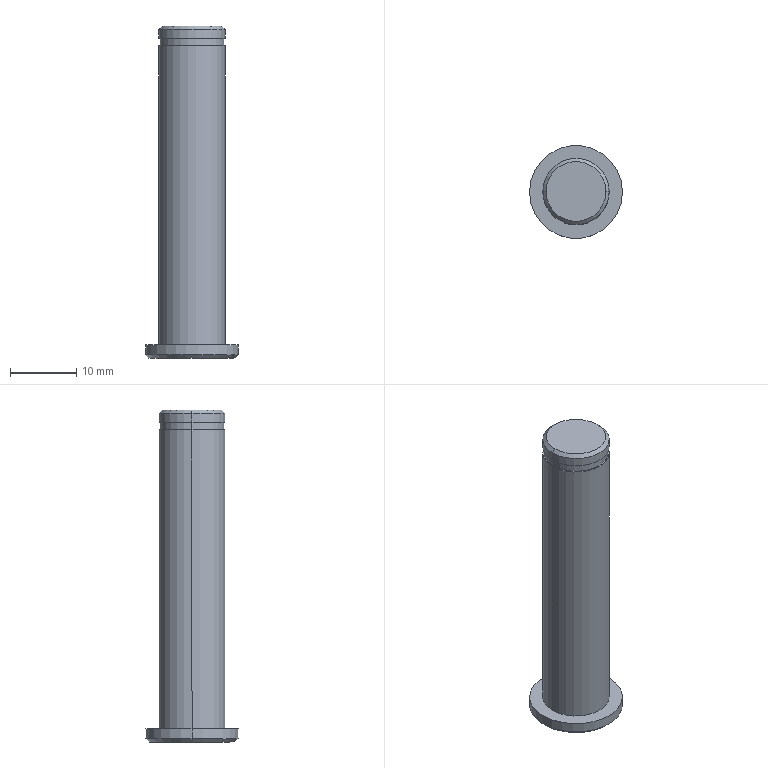Component | SolidWorks | RetainingRingPinMIC06_D10_L45-1 | 1 solid | 17 faces | box 14 x 14 x 50 mm | volume 4062 mm3 | cylinder 8 | plane 5 | cone 4 | commonest cylinder face diameters 10 x4 14 x2 9.6 x2
STEP:
#1=COLOUR_RGB('',0.7922,0.8196,0.9333);
#2=FILL_AREA_STYLE_COLOUR('',#1);
#3=FILL_AREA_STYLE('',(#2));
#4=SURFACE_STYLE_FILL_AREA(#3);
#5=SURFACE_SIDE_STYLE('',(#4));
#6=SURFACE_STYLE_USAGE(.BOTH.,#5);
#7=PRESENTATION_STYLE_ASSIGNMENT((#6));
#8=CARTESIAN_POINT('',(-0.07874,-0.9843,-0.8661));
#9=VERTEX_POINT('',#8);
#10=CARTESIAN_POINT('',(-0.07874,-0.9843,0.9055));
#11=VERTEX_POINT('',#10);
#12=CARTESIAN_POINT('',(-0.07874,-0.9843,-0.8661));
#13=DIRECTION('',(-0.,0.,1.));
#14=VECTOR('',#13,39.37);
#15=LINE('',#12,#14);
#16=EDGE_CURVE('',#9,#11,#15,.T.);
#17=ORIENTED_EDGE('',*,*,#16,.F.);
#18=CARTESIAN_POINT('',(0.315,-0.9843,-0.8661));
#19=VERTEX_POINT('',#18);
#20=CARTESIAN_POINT('',(0.1181,-0.9843,-0.8661));
#21=DIRECTION('',(-0.,0.,1.));
#22=DIRECTION('',(1.,0.,0.));
#23=AXIS2_PLACEMENT_3D('',#20,#21,#22);
#24=CIRCLE('',#23,0.1969);
#25=EDGE_CURVE('',#9,#19,#24,.T.);
#26=ORIENTED_EDGE('',*,*,#25,.T.);
#27=CARTESIAN_POINT('',(0.315,-0.9843,0.9055));
#28=VERTEX_POINT('',#27);
#29=CARTESIAN_POINT('',(0.315,-0.9843,-0.8661));
#30=DIRECTION('',(-0.,0.,1.));
#31=VECTOR('',#30,39.37);
#32=LINE('',#29,#31);
#33=EDGE_CURVE('',#19,#28,#32,.T.);
#34=ORIENTED_EDGE('',*,*,#33,.T.);
#35=CARTESIAN_POINT('',(0.1181,-0.9843,0.9055));
#36=DIRECTION('',(-0.,0.,1.));
#37=DIRECTION('',(1.,0.,0.));
#38=AXIS2_PLACEMENT_3D('',#35,#36,#37);
#39=CIRCLE('',#38,0.1969);
#40=EDGE_CURVE('',#11,#28,#39,.T.);
#41=ORIENTED_EDGE('',*,*,#40,.F.);
#42=EDGE_LOOP('',(#17,#26,#34,#41));
#43=FACE_OUTER_BOUND('',#42,.T.);
#44=CARTESIAN_POINT('',(0.1181,-0.9843,0.9055));
#45=DIRECTION('',(-0.,0.,1.));
#46=DIRECTION('',(-0.,1.,-0.));
#47=AXIS2_PLACEMENT_3D('',#44,#45,#46);
#48=CYLINDRICAL_SURFACE('',#47,0.1969);
#49=ADVANCED_FACE('',(#43),#48,.T.);
#50=CARTESIAN_POINT('',(-0.07087,-0.9843,0.9055));
#51=VERTEX_POINT('',#50);
#52=CARTESIAN_POINT('',(0.3071,-0.9843,0.9055));
#53=VERTEX_POINT('',#52);
#54=CARTESIAN_POINT('',(0.1181,-0.9843,0.9055));
#55=DIRECTION('',(-0.,0.,1.));
#56=DIRECTION('',(1.,0.,0.));
#57=AXIS2_PLACEMENT_3D('',#54,#55,#56);
#58=CIRCLE('',#57,0.189);
#59=EDGE_CURVE('',#51,#53,#58,.T.);
#60=ORIENTED_EDGE('',*,*,#59,.F.);
#61=CARTESIAN_POINT('',(0.1181,-0.9843,0.9055));
#62=DIRECTION('',(-0.,0.,1.));
#63=DIRECTION('',(1.,0.,0.));
#64=AXIS2_PLACEMENT_3D('',#61,#62,#63);
#65=CIRCLE('',#64,0.189);
#66=EDGE_CURVE('',#53,#51,#65,.T.);
#67=ORIENTED_EDGE('',*,*,#66,.F.);
#68=EDGE_LOOP('',(#60,#67));
#69=FACE_BOUND('',#68,.T.);
#70=CARTESIAN_POINT('',(0.1181,-0.9843,0.9055));
#71=DIRECTION('',(-0.,0.,1.));
#72=DIRECTION('',(1.,0.,0.));
#73=AXIS2_PLACEMENT_3D('',#70,#71,#72);
#74=CIRCLE('',#73,0.1969);
#75=EDGE_CURVE('',#28,#11,#74,.T.);
#76=ORIENTED_EDGE('',*,*,#75,.T.);
#77=ORIENTED_EDGE('',*,*,#40,.T.);
#78=EDGE_LOOP('',(#76,#77));
#79=FACE_OUTER_BOUND('',#78,.T.);
#80=CARTESIAN_POINT('',(0.1181,-0.7874,0.9055));
#81=DIRECTION('',(0.,-0.,-1.));
#82=DIRECTION('',(-1.,-0.,-0.));
#83=AXIS2_PLACEMENT_3D('',#80,#81,#82);
#84=PLANE('',#83);
#85=ADVANCED_FACE('',(#69,#79),#84,.F.);
#86=ORIENTED_EDGE('',*,*,#16,.T.);
#87=ORIENTED_EDGE('',*,*,#75,.F.);
#88=ORIENTED_EDGE('',*,*,#33,.F.);
#89=CARTESIAN_POINT('',(0.1181,-0.9843,-0.8661));
#90=DIRECTION('',(-0.,0.,1.));
#91=DIRECTION('',(1.,0.,0.));
#92=AXIS2_PLACEMENT_3D('',#89,#90,#91);
#93=CIRCLE('',#92,0.1969);
#94=EDGE_CURVE('',#19,#9,#93,.T.);
#95=ORIENTED_EDGE('',*,*,#94,.T.);
#96=EDGE_LOOP('',(#86,#87,#88,#95));
#97=FACE_OUTER_BOUND('',#96,.T.);
#98=CARTESIAN_POINT('',(0.1181,-0.9843,0.9055));
#99=DIRECTION('',(-0.,0.,1.));
#100=DIRECTION('',(0.,-1.,0.));
#101=AXIS2_PLACEMENT_3D('',#98,#99,#100);
#102=CYLINDRICAL_SURFACE('',#101,0.1969);
#103=ADVANCED_FACE('',(#97),#102,.T.);
#104=ORIENTED_EDGE('',*,*,#25,.F.);
#105=ORIENTED_EDGE('',*,*,#94,.F.);
#106=EDGE_LOOP('',(#104,#105));
#107=FACE_BOUND('',#106,.T.);
#108=CARTESIAN_POINT('',(0.3937,-0.9843,-0.8661));
#109=VERTEX_POINT('',#108);
#110=CARTESIAN_POINT('',(-0.1575,-0.9843,-0.8661));
#111=VERTEX_POINT('',#110);
#112=CARTESIAN_POINT('',(0.1181,-0.9843,-0.8661));
#113=DIRECTION('',(-0.,0.,1.));
#114=DIRECTION('',(1.,0.,0.));
#115=AXIS2_PLACEMENT_3D('',#112,#113,#114);
#116=CIRCLE('',#115,0.2756);
#117=EDGE_CURVE('',#109,#111,#116,.T.);
#118=ORIENTED_EDGE('',*,*,#117,.T.);
#119=CARTESIAN_POINT('',(0.1181,-0.9843,-0.8661));
#120=DIRECTION('',(-0.,0.,1.));
#121=DIRECTION('',(1.,0.,0.));
#122=AXIS2_PLACEMENT_3D('',#119,#120,#121);
#123=CIRCLE('',#122,0.2756);
#124=EDGE_CURVE('',#111,#109,#123,.T.);
#125=ORIENTED_EDGE('',*,*,#124,.T.);
#126=EDGE_LOOP('',(#118,#125));
#127=FACE_OUTER_BOUND('',#126,.T.);
#128=CARTESIAN_POINT('',(0.1181,-0.7087,-0.8661));
#129=DIRECTION('',(0.,-0.,-1.));
#130=DIRECTION('',(-1.,-0.,-0.));
#131=AXIS2_PLACEMENT_3D('',#128,#129,#130);
#132=PLANE('',#131);
#133=ADVANCED_FACE('',(#107,#127),#132,.F.);
#134=CARTESIAN_POINT('',(-0.1575,-0.9843,-0.9252));
#135=VERTEX_POINT('',#134);
#136=CARTESIAN_POINT('',(-0.1575,-0.9843,-0.9252));
#137=DIRECTION('',(-0.,0.,1.));
#138=VECTOR('',#137,39.37);
#139=LINE('',#136,#138);
#140=EDGE_CURVE('',#135,#111,#139,.T.);
#141=ORIENTED_EDGE('',*,*,#140,.F.);
#142=CARTESIAN_POINT('',(0.3937,-0.9843,-0.9252));
#143=VERTEX_POINT('',#142);
#144=CARTESIAN_POINT('',(0.1181,-0.9843,-0.9252));
#145=DIRECTION('',(-0.,0.,1.));
#146=DIRECTION('',(1.,0.,0.));
#147=AXIS2_PLACEMENT_3D('',#144,#145,#146);
#148=CIRCLE('',#147,0.2756);
#149=EDGE_CURVE('',#135,#143,#148,.T.);
#150=ORIENTED_EDGE('',*,*,#149,.T.);
#151=CARTESIAN_POINT('',(0.3937,-0.9843,-0.9252));
#152=DIRECTION('',(-0.,0.,1.));
#153=VECTOR('',#152,39.37);
#154=LINE('',#151,#153);
#155=EDGE_CURVE('',#143,#109,#154,.T.);
#156=ORIENTED_EDGE('',*,*,#155,.T.);
#157=ORIENTED_EDGE('',*,*,#124,.F.);
#158=EDGE_LOOP('',(#141,#150,#156,#157));
#159=FACE_OUTER_BOUND('',#158,.T.);
#160=CARTESIAN_POINT('',(0.1181,-0.9843,-0.8661));
#161=DIRECTION('',(-0.,0.,1.));
#162=DIRECTION('',(-0.,1.,-0.));
#163=AXIS2_PLACEMENT_3D('',#160,#161,#162);
#164=CYLINDRICAL_SURFACE('',#163,0.2756);
#165=ADVANCED_FACE('',(#159),#164,.T.);
#166=ORIENTED_EDGE('',*,*,#140,.T.);
#167=ORIENTED_EDGE('',*,*,#117,.F.);
#168=ORIENTED_EDGE('',*,*,#155,.F.);
#169=CARTESIAN_POINT('',(0.1181,-0.9843,-0.9252));
#170=DIRECTION('',(-0.,0.,1.));
#171=DIRECTION('',(1.,0.,0.));
#172=AXIS2_PLACEMENT_3D('',#169,#170,#171);
#173=CIRCLE('',#172,0.2756);
#174=EDGE_CURVE('',#143,#135,#173,.T.);
#175=ORIENTED_EDGE('',*,*,#174,.T.);
#176=EDGE_LOOP('',(#166,#167,#168,#175));
#177=FACE_OUTER_BOUND('',#176,.T.);
#178=CARTESIAN_POINT('',(0.1181,-0.9843,-0.8661));
#179=DIRECTION('',(-0.,0.,1.));
#180=DIRECTION('',(0.,-1.,0.));
#181=AXIS2_PLACEMENT_3D('',#178,#179,#180);
#182=CYLINDRICAL_SURFACE('',#181,0.2756);
#183=ADVANCED_FACE('',(#177),#182,.T.);
#184=CARTESIAN_POINT('',(-0.1378,-0.9843,-0.9449));
#185=VERTEX_POINT('',#184);
#186=CARTESIAN_POINT('',(-0.1378,-0.9843,-0.9449));
#187=DIRECTION('',(-0.7071,0.,0.7071));
#188=VECTOR('',#187,39.37);
#189=LINE('',#186,#188);
#190=EDGE_CURVE('',#185,#135,#189,.T.);
#191=ORIENTED_EDGE('',*,*,#190,.T.);
#192=ORIENTED_EDGE('',*,*,#174,.F.);
#193=CARTESIAN_POINT('',(0.374,-0.9843,-0.9449));
#194=VERTEX_POINT('',#193);
#195=CARTESIAN_POINT('',(0.374,-0.9843,-0.9449));
#196=DIRECTION('',(0.7071,0.,0.7071));
#197=VECTOR('',#196,39.37);
#198=LINE('',#195,#197);
#199=EDGE_CURVE('',#194,#143,#198,.T.);
#200=ORIENTED_EDGE('',*,*,#199,.F.);
#201=CARTESIAN_POINT('',(0.1181,-0.9843,-0.9449));
#202=DIRECTION('',(-0.,0.,1.));
#203=DIRECTION('',(1.,0.,0.));
#204=AXIS2_PLACEMENT_3D('',#201,#202,#203);
#205=CIRCLE('',#204,0.2559);
#206=EDGE_CURVE('',#194,#185,#205,.T.);
#207=ORIENTED_EDGE('',*,*,#206,.T.);
#208=EDGE_LOOP('',(#191,#192,#200,#207));
#209=FACE_OUTER_BOUND('',#208,.T.);
#210=CARTESIAN_POINT('',(0.1181,-0.9843,-0.9449));
#211=DIRECTION('',(-0.,0.,1.));
#212=DIRECTION('',(0.,-1.,0.));
#213=AXIS2_PLACEMENT_3D('',#210,#211,#212);
#214=CONICAL_SURFACE('',#213,0.2559,0.7854);
#215=ADVANCED_FACE('',(#209),#214,.T.);
#216=CARTESIAN_POINT('',(0.1181,-0.9843,-0.9449));
#217=DIRECTION('',(-0.,0.,1.));
#218=DIRECTION('',(1.,0.,0.));
#219=AXIS2_PLACEMENT_3D('',#216,#217,#218);
#220=CIRCLE('',#219,0.2559);
#221=EDGE_CURVE('',#185,#194,#220,.T.);
#222=ORIENTED_EDGE('',*,*,#221,.F.);
#223=ORIENTED_EDGE('',*,*,#206,.F.);
#224=EDGE_LOOP('',(#222,#223));
#225=FACE_OUTER_BOUND('',#224,.T.);
#226=CARTESIAN_POINT('',(0.1181,-0.9843,-0.9449));
#227=DIRECTION('',(-0.,0.,1.));
#228=DIRECTION('',(1.,0.,0.));
#229=AXIS2_PLACEMENT_3D('',#226,#227,#228);
#230=PLANE('',#229);
#231=ADVANCED_FACE('',(#225),#230,.F.);
#232=ORIENTED_EDGE('',*,*,#190,.F.);
#233=ORIENTED_EDGE('',*,*,#221,.T.);
#234=ORIENTED_EDGE('',*,*,#199,.T.);
#235=ORIENTED_EDGE('',*,*,#149,.F.);
#236=EDGE_LOOP('',(#232,#233,#234,#235));
#237=FACE_OUTER_BOUND('',#236,.T.);
#238=CARTESIAN_POINT('',(0.1181,-0.9843,-0.9449));
#239=DIRECTION('',(-0.,0.,1.));
#240=DIRECTION('',(-0.,1.,-0.));
#241=AXIS2_PLACEMENT_3D('',#238,#239,#240);
#242=CONICAL_SURFACE('',#241,0.2559,0.7854);
#243=ADVANCED_FACE('',(#237),#242,.T.);
#244=CARTESIAN_POINT('',(-0.07087,-0.9843,0.9508));
#245=VERTEX_POINT('',#244);
#246=CARTESIAN_POINT('',(-0.07087,-0.9843,0.9055));
#247=DIRECTION('',(-0.,0.,1.));
#248=VECTOR('',#247,39.37);
#249=LINE('',#246,#248);
#250=EDGE_CURVE('',#51,#245,#249,.T.);
#251=ORIENTED_EDGE('',*,*,#250,.T.);
#252=CARTESIAN_POINT('',(0.3071,-0.9843,0.9508));
#253=VERTEX_POINT('',#252);
#254=CARTESIAN_POINT('',(0.1181,-0.9843,0.9508));
#255=DIRECTION('',(-0.,0.,1.));
#256=DIRECTION('',(1.,0.,0.));
#257=AXIS2_PLACEMENT_3D('',#254,#255,#256);
#258=CIRCLE('',#257,0.189);
#259=EDGE_CURVE('',#253,#245,#258,.T.);
#260=ORIENTED_EDGE('',*,*,#259,.F.);
#261=CARTESIAN_POINT('',(0.3071,-0.9843,0.9055));
#262=DIRECTION('',(-0.,0.,1.));
#263=VECTOR('',#262,39.37);
#264=LINE('',#261,#263);
#265=EDGE_CURVE('',#53,#253,#264,.T.);
#266=ORIENTED_EDGE('',*,*,#265,.F.);
#267=ORIENTED_EDGE('',*,*,#66,.T.);
#268=EDGE_LOOP('',(#251,#260,#266,#267));
#269=FACE_OUTER_BOUND('',#268,.T.);
#270=CARTESIAN_POINT('',(0.1181,-0.9843,1.024));
#271=DIRECTION('',(-0.,0.,1.));
#272=DIRECTION('',(0.,-1.,0.));
#273=AXIS2_PLACEMENT_3D('',#270,#271,#272);
#274=CYLINDRICAL_SURFACE('',#273,0.189);
#275=ADVANCED_FACE('',(#269),#274,.T.);
#276=ORIENTED_EDGE('',*,*,#250,.F.);
#277=ORIENTED_EDGE('',*,*,#59,.T.);
#278=ORIENTED_EDGE('',*,*,#265,.T.);
#279=CARTESIAN_POINT('',(0.1181,-0.9843,0.9508));
#280=DIRECTION('',(-0.,0.,1.));
#281=DIRECTION('',(1.,0.,0.));
#282=AXIS2_PLACEMENT_3D('',#279,#280,#281);
#283=CIRCLE('',#282,0.189);
#284=EDGE_CURVE('',#245,#253,#283,.T.);
#285=ORIENTED_EDGE('',*,*,#284,.F.);
#286=EDGE_LOOP('',(#276,#277,#278,#285));
#287=FACE_OUTER_BOUND('',#286,.T.);
#288=CARTESIAN_POINT('',(0.1181,-0.9843,1.024));
#289=DIRECTION('',(-0.,0.,1.));
#290=DIRECTION('',(-0.,1.,-0.));
#291=AXIS2_PLACEMENT_3D('',#288,#289,#290);
#292=CYLINDRICAL_SURFACE('',#291,0.189);
#293=ADVANCED_FACE('',(#287),#292,.T.);
#294=CARTESIAN_POINT('',(-0.07874,-0.9843,0.9508));
#295=VERTEX_POINT('',#294);
#296=CARTESIAN_POINT('',(0.315,-0.9843,0.9508));
#297=VERTEX_POINT('',#296);
#298=CARTESIAN_POINT('',(0.1181,-0.9843,0.9508));
#299=DIRECTION('',(-0.,0.,1.));
#300=DIRECTION('',(1.,0.,0.));
#301=AXIS2_PLACEMENT_3D('',#298,#299,#300);
#302=CIRCLE('',#301,0.1969);
#303=EDGE_CURVE('',#295,#297,#302,.T.);
#304=ORIENTED_EDGE('',*,*,#303,.F.);
#305=CARTESIAN_POINT('',(0.1181,-0.9843,0.9508));
#306=DIRECTION('',(-0.,0.,1.));
#307=DIRECTION('',(1.,0.,0.));
#308=AXIS2_PLACEMENT_3D('',#305,#306,#307);
#309=CIRCLE('',#308,0.1969);
#310=EDGE_CURVE('',#297,#295,#309,.T.);
#311=ORIENTED_EDGE('',*,*,#310,.F.);
#312=EDGE_LOOP('',(#304,#311));
#313=FACE_OUTER_BOUND('',#312,.T.);
#314=ORIENTED_EDGE('',*,*,#259,.T.);
#315=ORIENTED_EDGE('',*,*,#284,.T.);
#316=EDGE_LOOP('',(#314,#315));
#317=FACE_BOUND('',#316,.T.);
#318=CARTESIAN_POINT('',(0.1181,-0.7953,0.9508));
#319=DIRECTION('',(-0.,0.,1.));
#320=DIRECTION('',(1.,0.,0.));
#321=AXIS2_PLACEMENT_3D('',#318,#319,#320);
#322=PLANE('',#321);
#323=ADVANCED_FACE('',(#313,#317),#322,.F.);
#324=CARTESIAN_POINT('',(-0.07874,-0.9843,1.004));
#325=VERTEX_POINT('',#324);
#326=CARTESIAN_POINT('',(-0.07874,-0.9843,0.9508));
#327=DIRECTION('',(-0.,0.,1.));
#328=VECTOR('',#327,39.37);
#329=LINE('',#326,#328);
#330=EDGE_CURVE('',#295,#325,#329,.T.);
#331=ORIENTED_EDGE('',*,*,#330,.T.);
#332=CARTESIAN_POINT('',(0.315,-0.9843,1.004));
#333=VERTEX_POINT('',#332);
#334=CARTESIAN_POINT('',(0.1181,-0.9843,1.004));
#335=DIRECTION('',(-0.,0.,1.));
#336=DIRECTION('',(1.,0.,0.));
#337=AXIS2_PLACEMENT_3D('',#334,#335,#336);
#338=CIRCLE('',#337,0.1969);
#339=EDGE_CURVE('',#333,#325,#338,.T.);
#340=ORIENTED_EDGE('',*,*,#339,.F.);
#341=CARTESIAN_POINT('',(0.315,-0.9843,0.9508));
#342=DIRECTION('',(-0.,0.,1.));
#343=VECTOR('',#342,39.37);
#344=LINE('',#341,#343);
#345=EDGE_CURVE('',#297,#333,#344,.T.);
#346=ORIENTED_EDGE('',*,*,#345,.F.);
#347=ORIENTED_EDGE('',*,*,#310,.T.);
#348=EDGE_LOOP('',(#331,#340,#346,#347));
#349=FACE_OUTER_BOUND('',#348,.T.);
#350=CARTESIAN_POINT('',(0.1181,-0.9843,1.024));
#351=DIRECTION('',(-0.,0.,1.));
#352=DIRECTION('',(0.,-1.,0.));
#353=AXIS2_PLACEMENT_3D('',#350,#351,#352);
#354=CYLINDRICAL_SURFACE('',#353,0.1969);
#355=ADVANCED_FACE('',(#349),#354,.T.);
#356=ORIENTED_EDGE('',*,*,#330,.F.);
#357=ORIENTED_EDGE('',*,*,#303,.T.);
#358=ORIENTED_EDGE('',*,*,#345,.T.);
#359=CARTESIAN_POINT('',(0.1181,-0.9843,1.004));
#360=DIRECTION('',(-0.,0.,1.));
#361=DIRECTION('',(1.,0.,0.));
#362=AXIS2_PLACEMENT_3D('',#359,#360,#361);
#363=CIRCLE('',#362,0.1969);
#364=EDGE_CURVE('',#325,#333,#363,.T.);
#365=ORIENTED_EDGE('',*,*,#364,.F.);
#366=EDGE_LOOP('',(#356,#357,#358,#365));
#367=FACE_OUTER_BOUND('',#366,.T.);
#368=CARTESIAN_POINT('',(0.1181,-0.9843,1.024));
#369=DIRECTION('',(-0.,0.,1.));
#370=DIRECTION('',(-0.,1.,-0.));
#371=AXIS2_PLACEMENT_3D('',#368,#369,#370);
#372=CYLINDRICAL_SURFACE('',#371,0.1969);
#373=ADVANCED_FACE('',(#367),#372,.T.);
#374=CARTESIAN_POINT('',(0.2953,-0.9843,1.024));
#375=VERTEX_POINT('',#374);
#376=CARTESIAN_POINT('',(0.2953,-0.9843,1.024));
#377=DIRECTION('',(0.7071,0.,-0.7071));
#378=VECTOR('',#377,39.37);
#379=LINE('',#376,#378);
#380=EDGE_CURVE('',#375,#333,#379,.T.);
#381=ORIENTED_EDGE('',*,*,#380,.F.);
#382=CARTESIAN_POINT('',(-0.05906,-0.9843,1.024));
#383=VERTEX_POINT('',#382);
#384=CARTESIAN_POINT('',(0.1181,-0.9843,1.024));
#385=DIRECTION('',(-0.,0.,1.));
#386=DIRECTION('',(1.,0.,0.));
#387=AXIS2_PLACEMENT_3D('',#384,#385,#386);
#388=CIRCLE('',#387,0.1772);
#389=EDGE_CURVE('',#383,#375,#388,.T.);
#390=ORIENTED_EDGE('',*,*,#389,.F.);
#391=CARTESIAN_POINT('',(-0.05906,-0.9843,1.024));
#392=DIRECTION('',(-0.7071,-0.,-0.7071));
#393=VECTOR('',#392,39.37);
#394=LINE('',#391,#393);
#395=EDGE_CURVE('',#383,#325,#394,.T.);
#396=ORIENTED_EDGE('',*,*,#395,.T.);
#397=ORIENTED_EDGE('',*,*,#364,.T.);
#398=EDGE_LOOP('',(#381,#390,#396,#397));
#399=FACE_OUTER_BOUND('',#398,.T.);
#400=CARTESIAN_POINT('',(0.1181,-0.9843,1.004));
#401=DIRECTION('',(0.,-0.,-1.));
#402=DIRECTION('',(-0.,1.,-0.));
#403=AXIS2_PLACEMENT_3D('',#400,#401,#402);
#404=CONICAL_SURFACE('',#403,0.1969,0.7854);
#405=ADVANCED_FACE('',(#399),#404,.T.);
#406=ORIENTED_EDGE('',*,*,#380,.T.);
#407=ORIENTED_EDGE('',*,*,#339,.T.);
#408=ORIENTED_EDGE('',*,*,#395,.F.);
#409=CARTESIAN_POINT('',(0.1181,-0.9843,1.024));
#410=DIRECTION('',(-0.,0.,1.));
#411=DIRECTION('',(1.,0.,0.));
#412=AXIS2_PLACEMENT_3D('',#409,#410,#411);
#413=CIRCLE('',#412,0.1772);
#414=EDGE_CURVE('',#375,#383,#413,.T.);
#415=ORIENTED_EDGE('',*,*,#414,.F.);
#416=EDGE_LOOP('',(#406,#407,#408,#415));
#417=FACE_OUTER_BOUND('',#416,.T.);
#418=CARTESIAN_POINT('',(0.1181,-0.9843,1.004));
#419=DIRECTION('',(0.,-0.,-1.));
#420=DIRECTION('',(0.,-1.,0.));
#421=AXIS2_PLACEMENT_3D('',#418,#419,#420);
#422=CONICAL_SURFACE('',#421,0.1969,0.7854);
#423=ADVANCED_FACE('',(#417),#422,.T.);
#424=ORIENTED_EDGE('',*,*,#414,.T.);
#425=ORIENTED_EDGE('',*,*,#389,.T.);
#426=EDGE_LOOP('',(#424,#425));
#427=FACE_OUTER_BOUND('',#426,.T.);
#428=CARTESIAN_POINT('',(0.1181,-0.8071,1.024));
#429=DIRECTION('',(0.,-0.,-1.));
#430=DIRECTION('',(-1.,-0.,-0.));
#431=AXIS2_PLACEMENT_3D('',#428,#429,#430);
#432=PLANE('',#431);
#433=ADVANCED_FACE('',(#427),#432,.F.);
#434=CLOSED_SHELL('',(#49,#85,#103,#133,#165,#183,#215,#231,#243,#275,#293,#323,#355,#373,#405,#423,#433));
#435=MANIFOLD_SOLID_BREP('',#434);
#436=STYLED_ITEM('',(#7),#435);
#437=(LENGTH_UNIT()NAMED_UNIT(*)SI_UNIT($,.METRE.));
#438=LENGTH_MEASURE_WITH_UNIT(LENGTH_MEASURE(0.0254),#437);
#439=DIMENSIONAL_EXPONENTS(1.,0.,0.,0.,0.,0.,0.);
#440=(CONVERSION_BASED_UNIT('',#438)LENGTH_UNIT()NAMED_UNIT(#439));
#441=UNCERTAINTY_MEASURE_WITH_UNIT(LENGTH_MEASURE(0.00001),#440,'','');
#442=(NAMED_UNIT(*)PLANE_ANGLE_UNIT()SI_UNIT($,.RADIAN.));
#443=(NAMED_UNIT(*)SI_UNIT($,.STERADIAN.)SOLID_ANGLE_UNIT());
#444=(GEOMETRIC_REPRESENTATION_CONTEXT(3)GLOBAL_UNCERTAINTY_ASSIGNED_CONTEXT((#441))GLOBAL_UNIT_ASSIGNED_CONTEXT((#440,#442,#443))REPRESENTATION_CONTEXT('',''));
#445=MECHANICAL_DESIGN_GEOMETRIC_PRESENTATION_REPRESENTATION('',(#436),#444);
#446=CARTESIAN_POINT('',(0.,0.,0.));
#447=DIRECTION('',(0.,0.,1.));
#448=DIRECTION('',(1.,0.,0.));
#449=AXIS2_PLACEMENT_3D('',#446,#447,#448);
#450=(LENGTH_UNIT()NAMED_UNIT(*)SI_UNIT($,.METRE.));
#451=LENGTH_MEASURE_WITH_UNIT(LENGTH_MEASURE(0.0254),#450);
#452=DIMENSIONAL_EXPONENTS(1.,0.,0.,0.,0.,0.,0.);
#453=(CONVERSION_BASED_UNIT('',#451)LENGTH_UNIT()NAMED_UNIT(#452));
#454=UNCERTAINTY_MEASURE_WITH_UNIT(LENGTH_MEASURE(0.00001),#453,'','');
#455=(NAMED_UNIT(*)PLANE_ANGLE_UNIT()SI_UNIT($,.RADIAN.));
#456=(NAMED_UNIT(*)SI_UNIT($,.STERADIAN.)SOLID_ANGLE_UNIT());
#457=(GEOMETRIC_REPRESENTATION_CONTEXT(3)GLOBAL_UNCERTAINTY_ASSIGNED_CONTEXT((#454))GLOBAL_UNIT_ASSIGNED_CONTEXT((#453,#455,#456))REPRESENTATION_CONTEXT('',''));
#458=ADVANCED_BREP_SHAPE_REPRESENTATION('',(#435,#449),#457);
#459=PRESENTATION_LAYER_ASSIGNMENT('','',(#436));